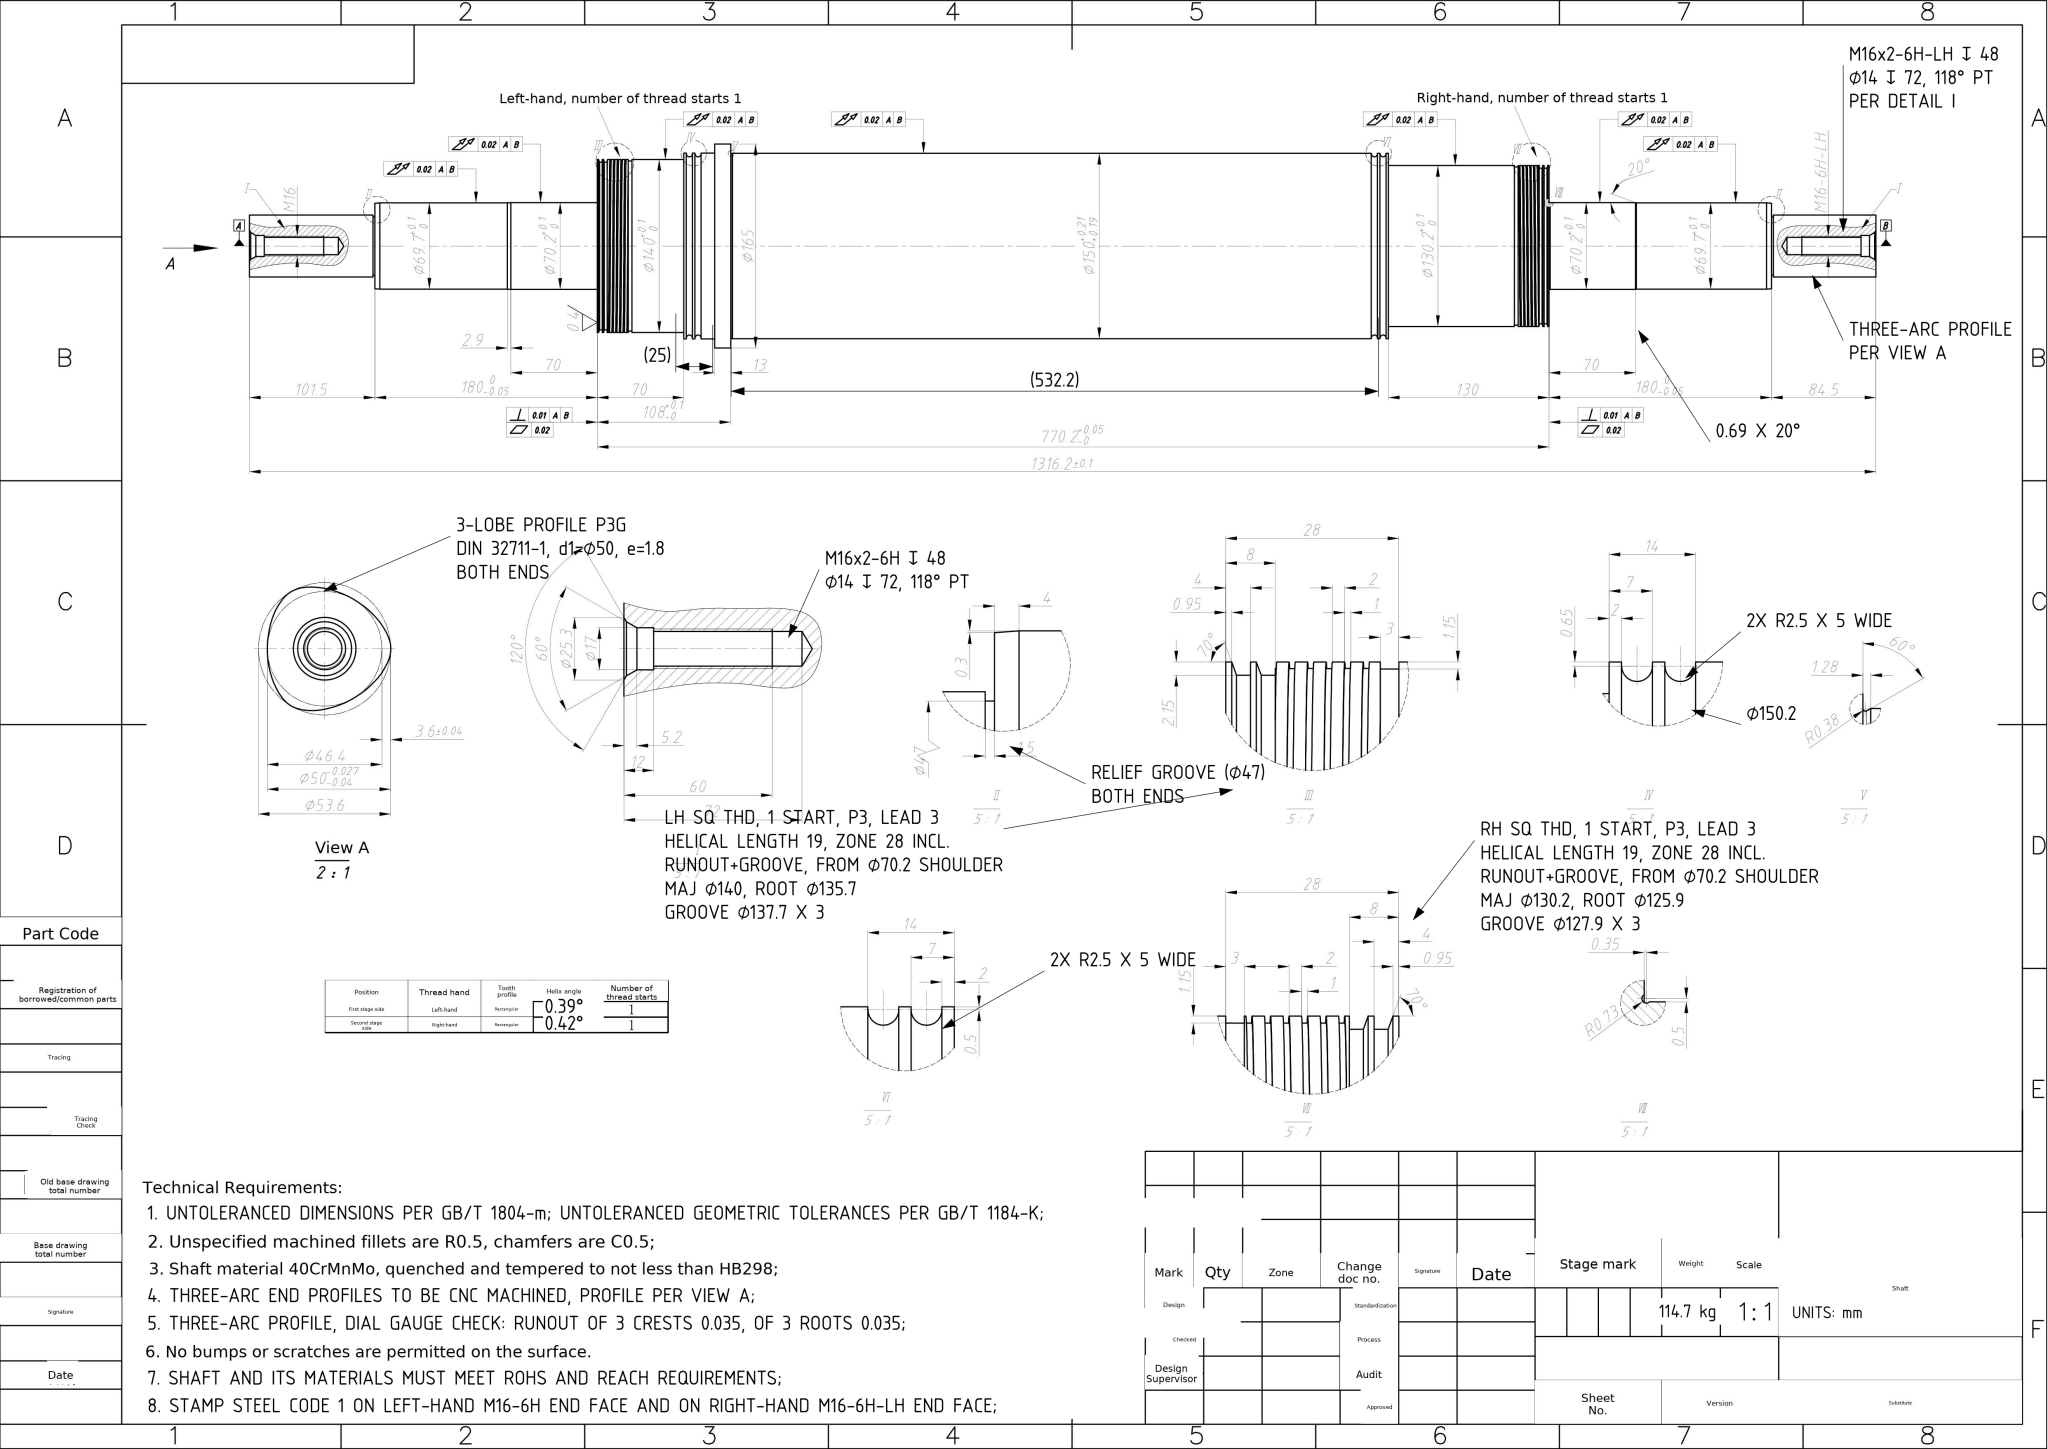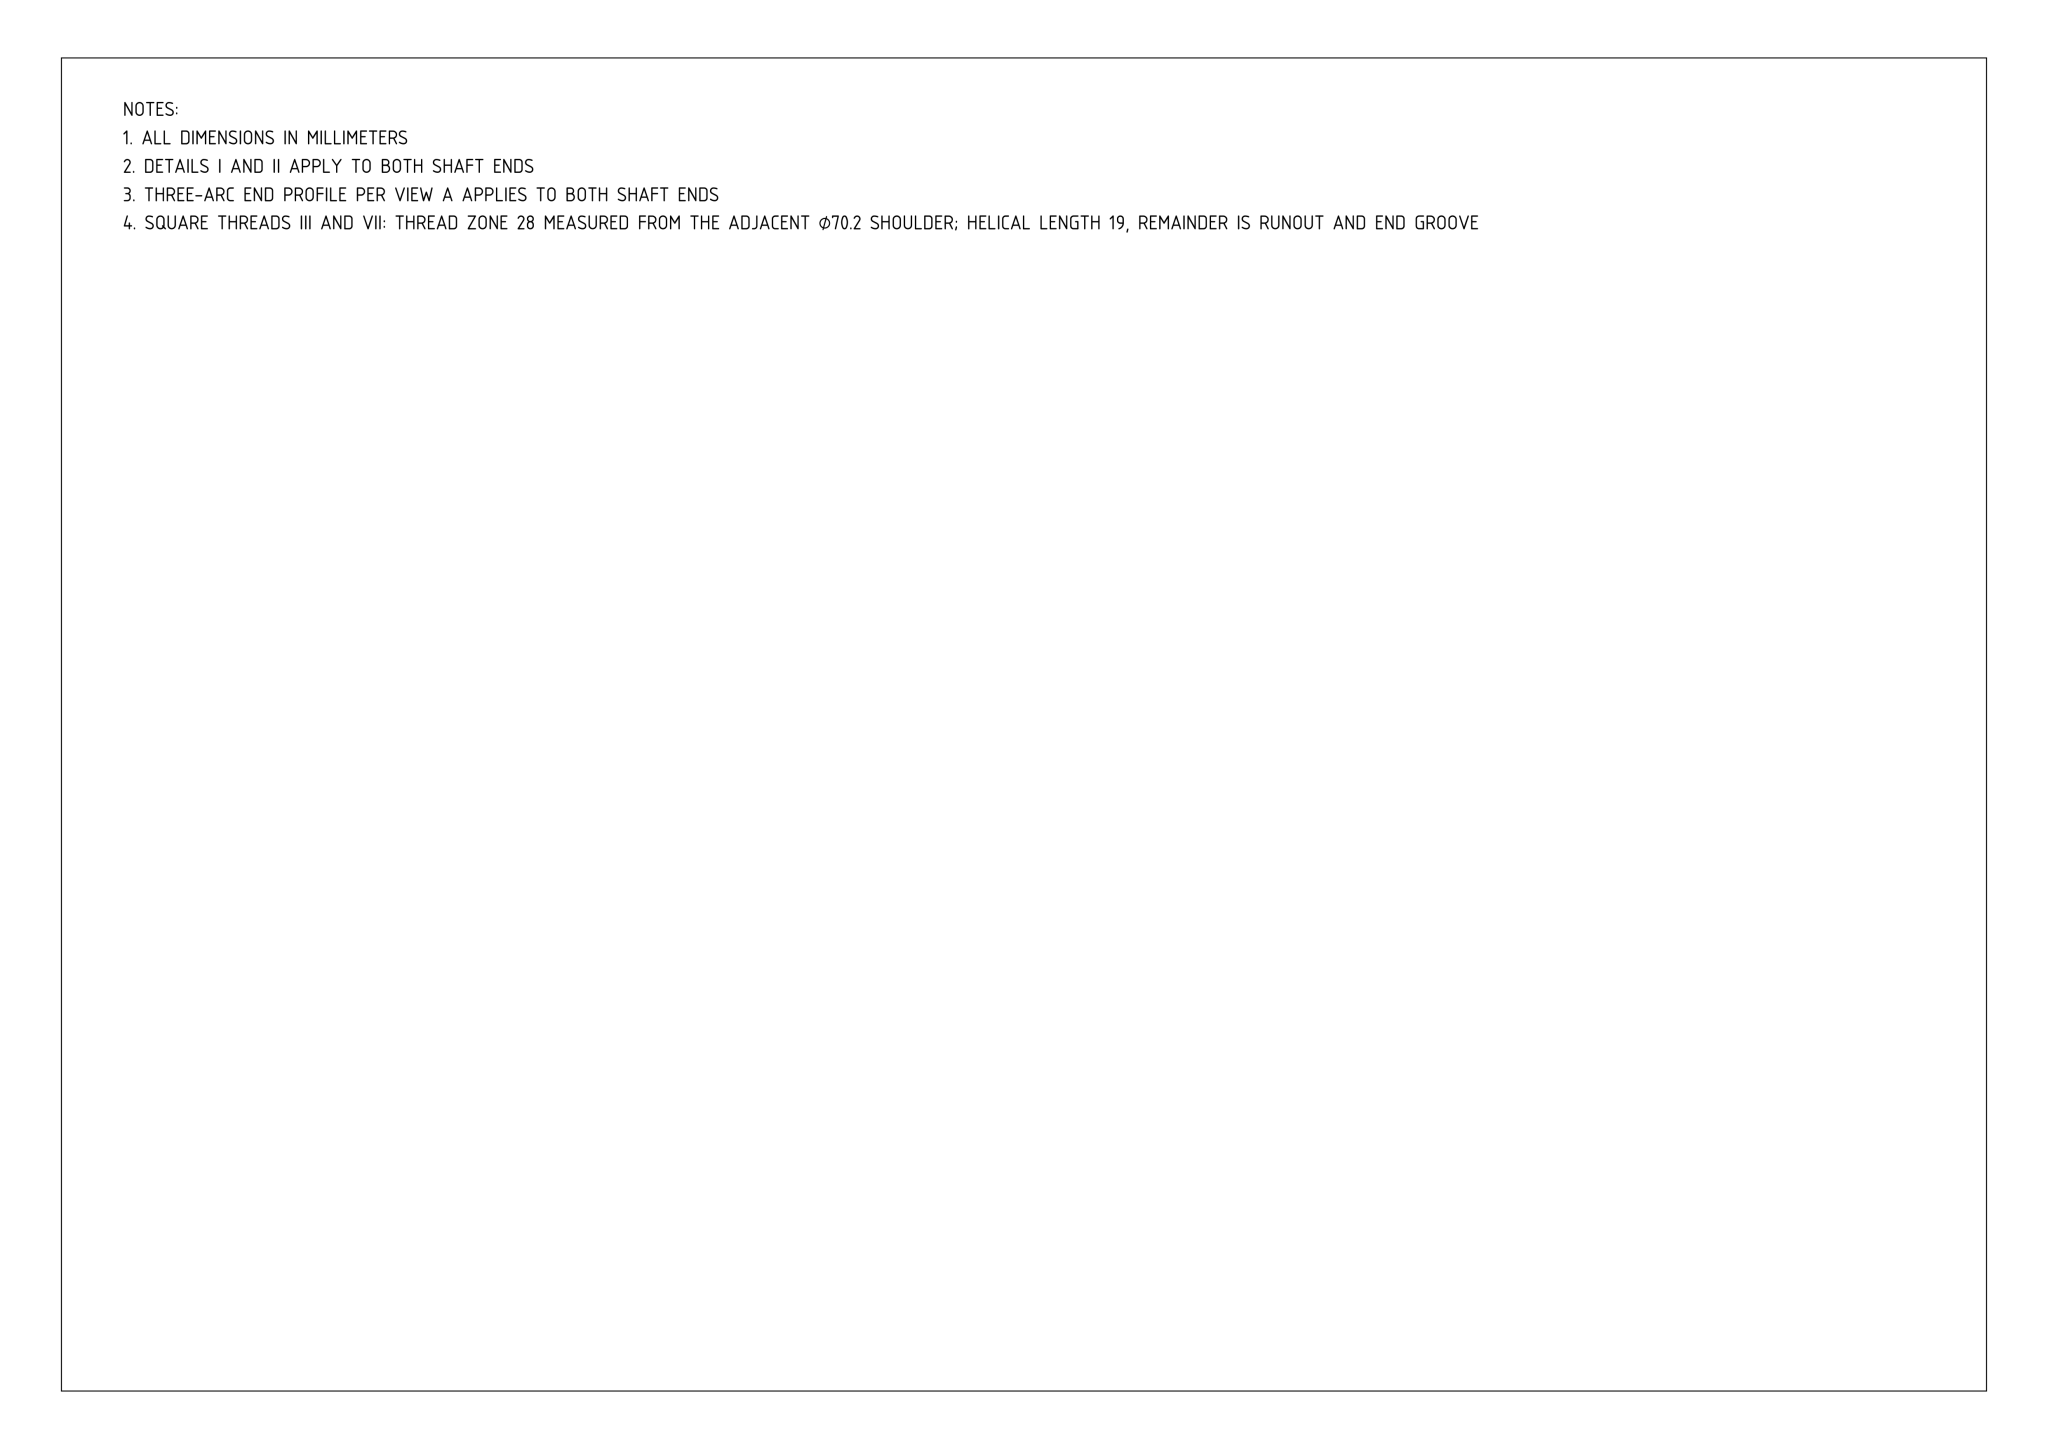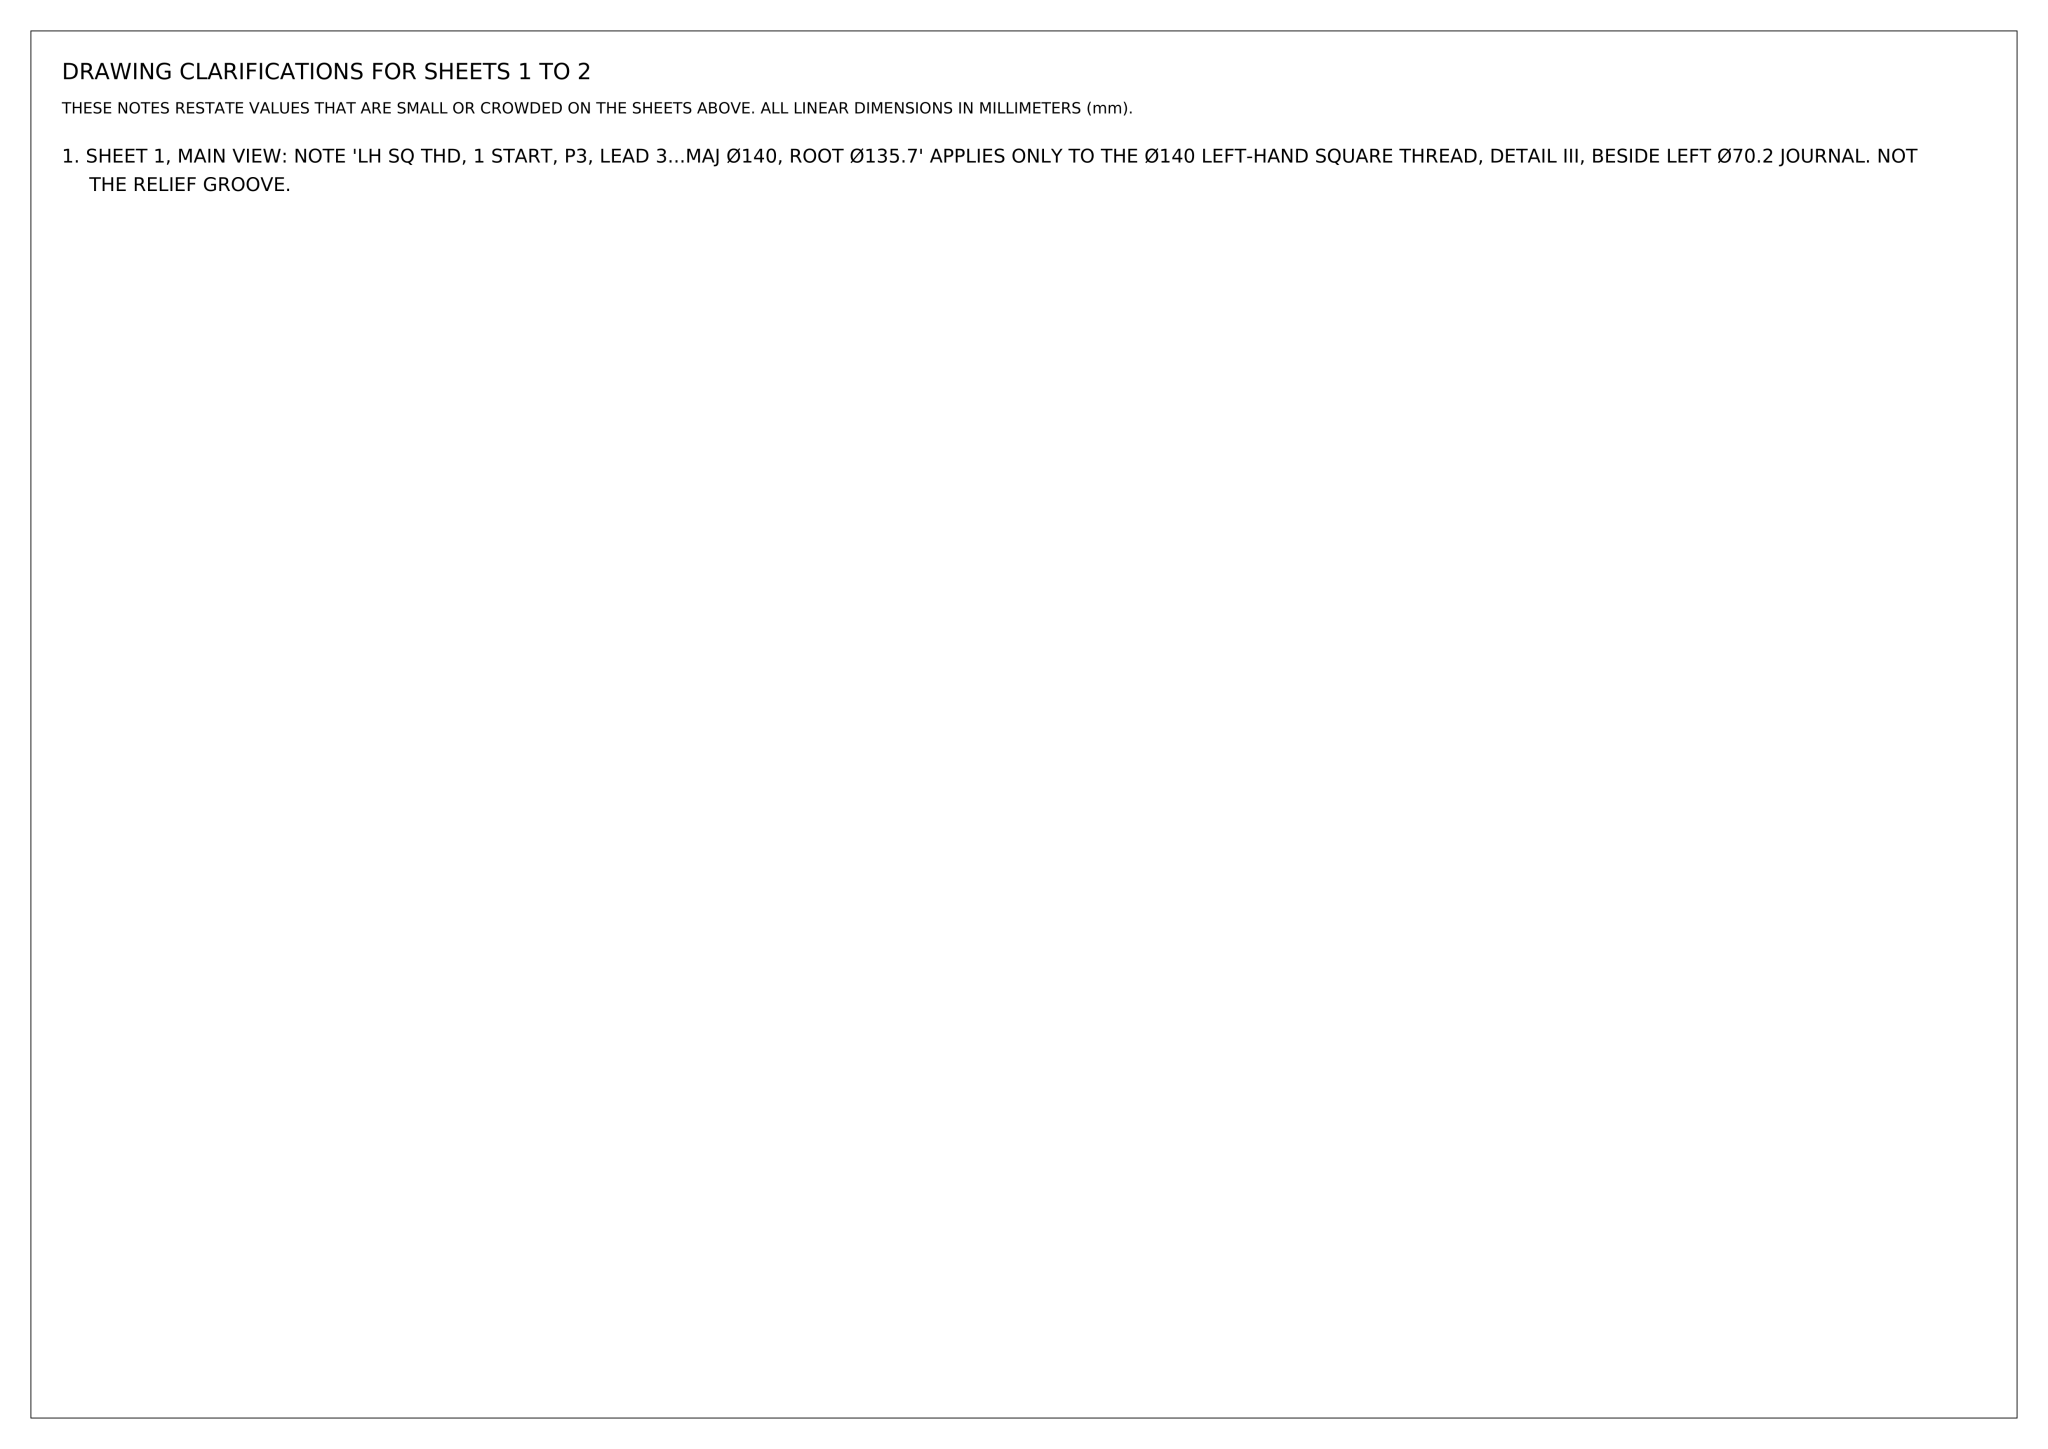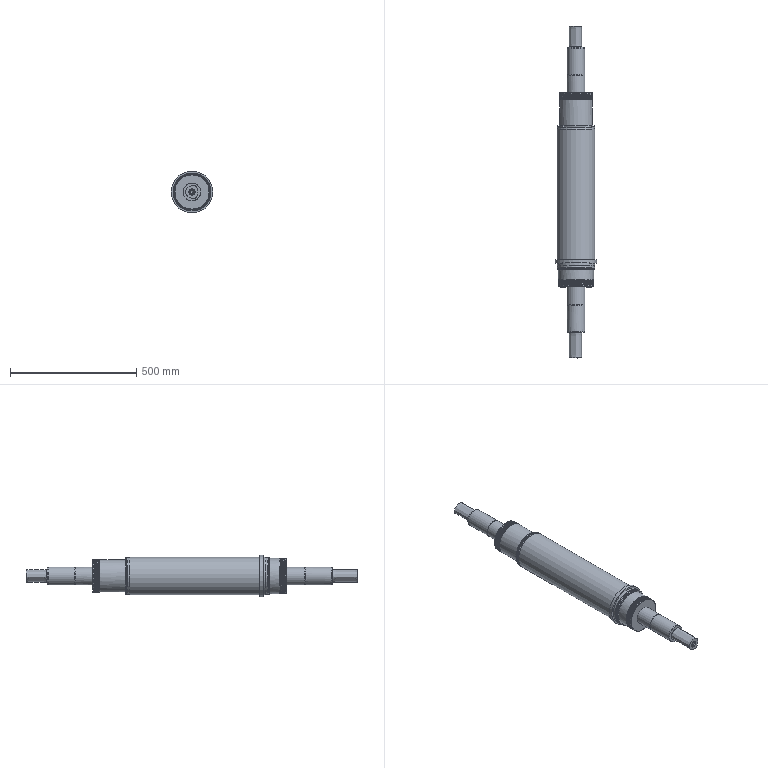Part | NX | mm | 1 solid | 100 faces | box 165 x 1316.2 x 165 mm | volume 14606488 mm3 | plane 40 | cylinder 31 | cone 15 | torus 6 | spline 6 | other 2 | commonest cylinder face diameters 130.2 x4 140 x4 150.2 x3 150 x3 70.2 x2 69.7 x2 135.7 x2 125.9 x2